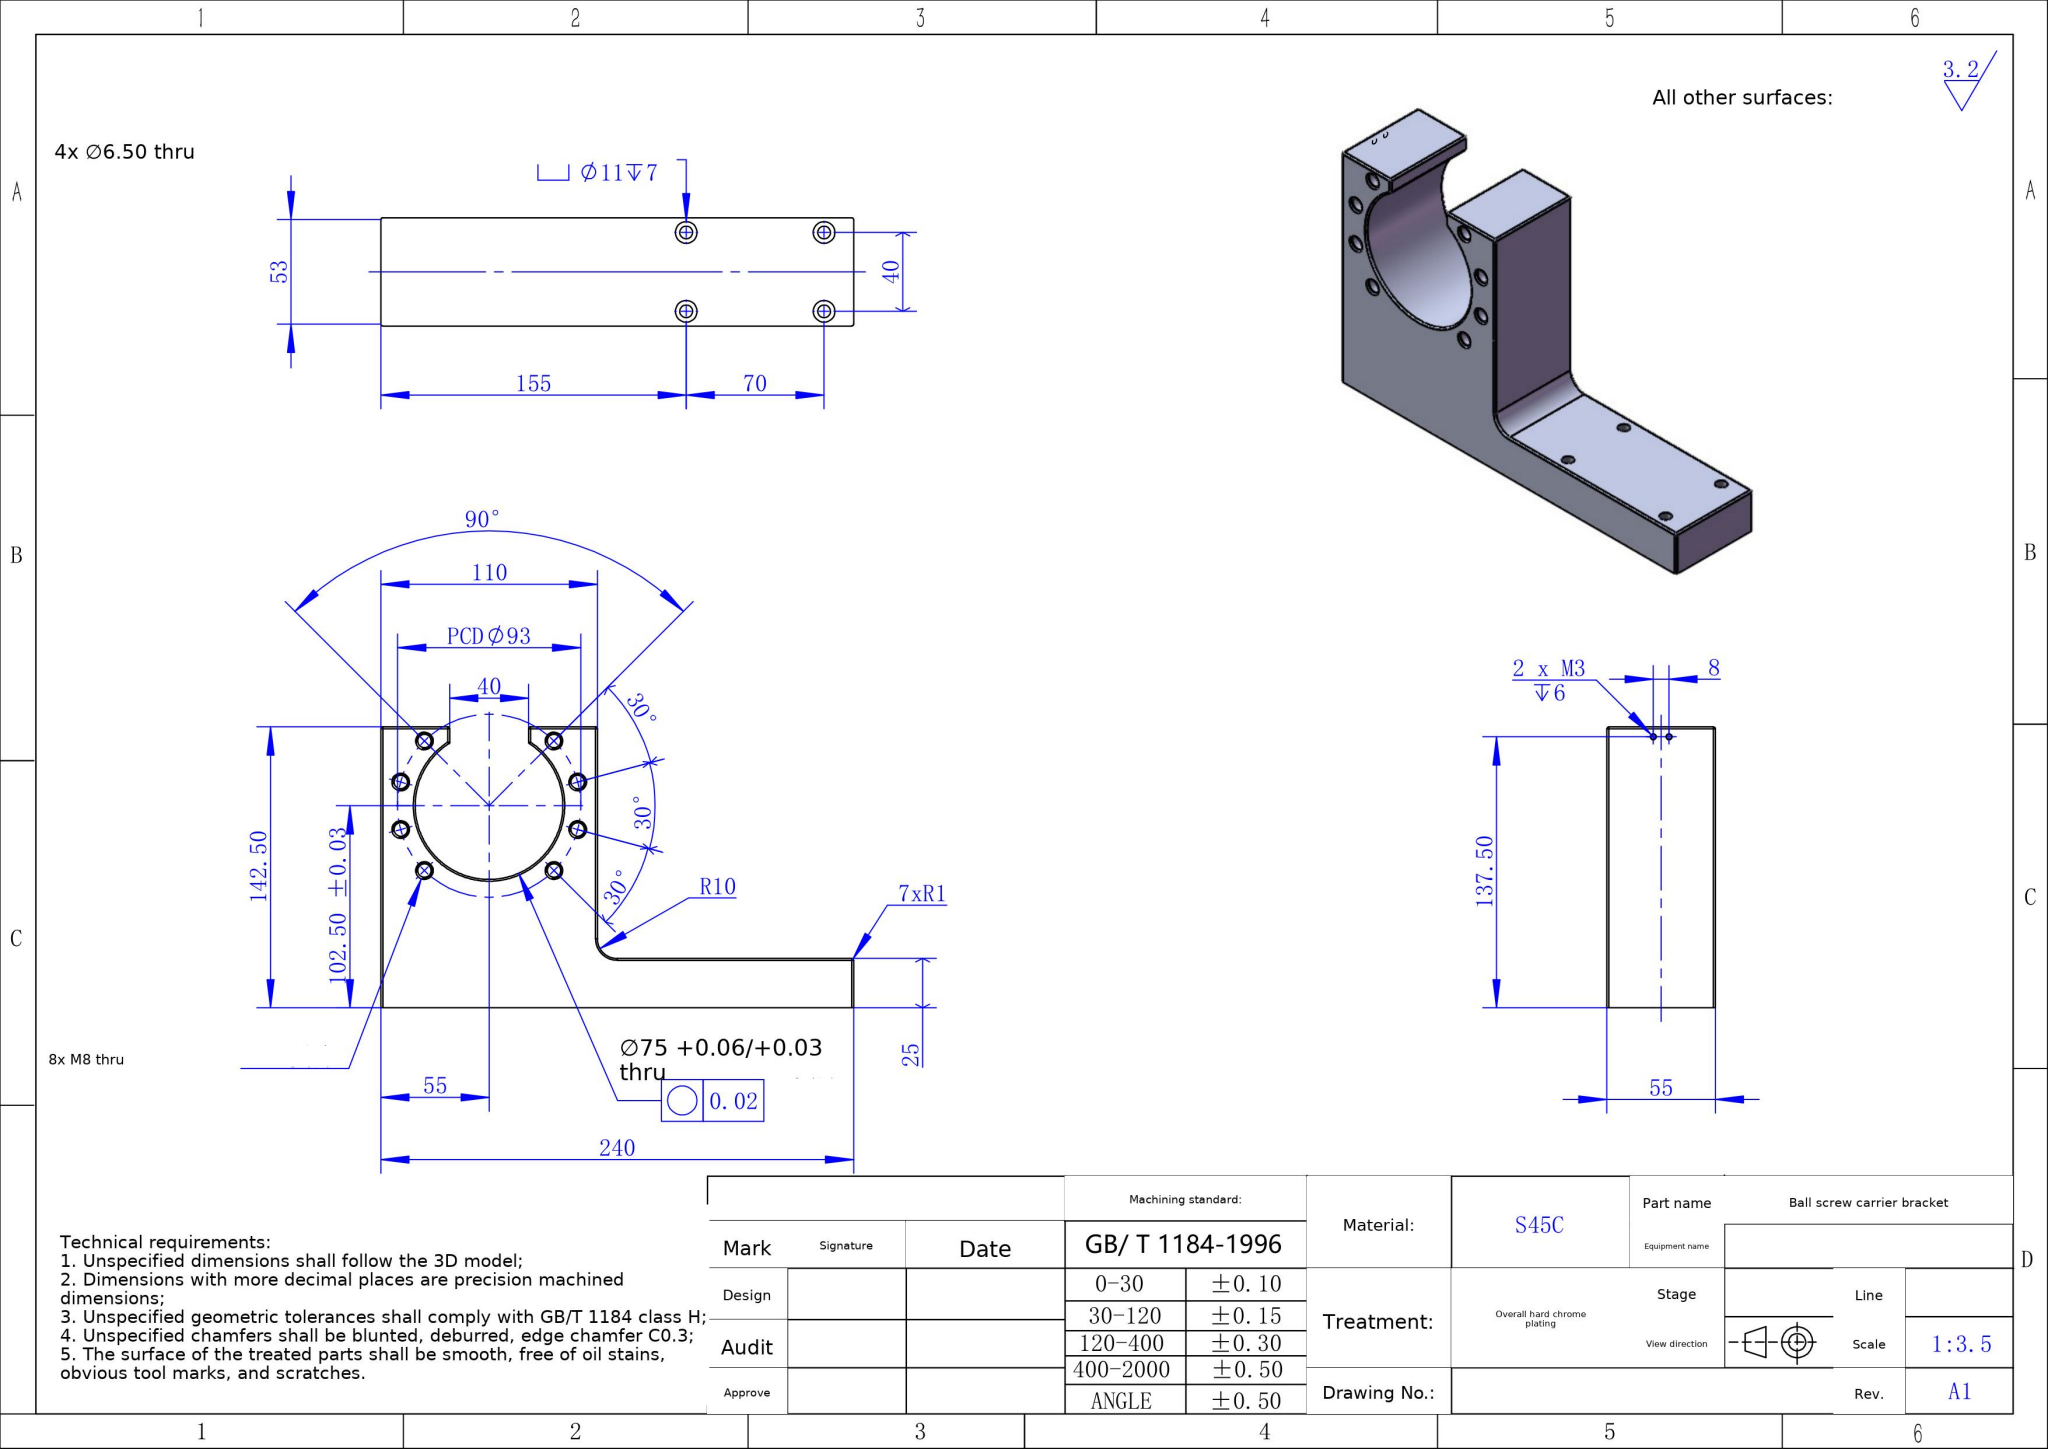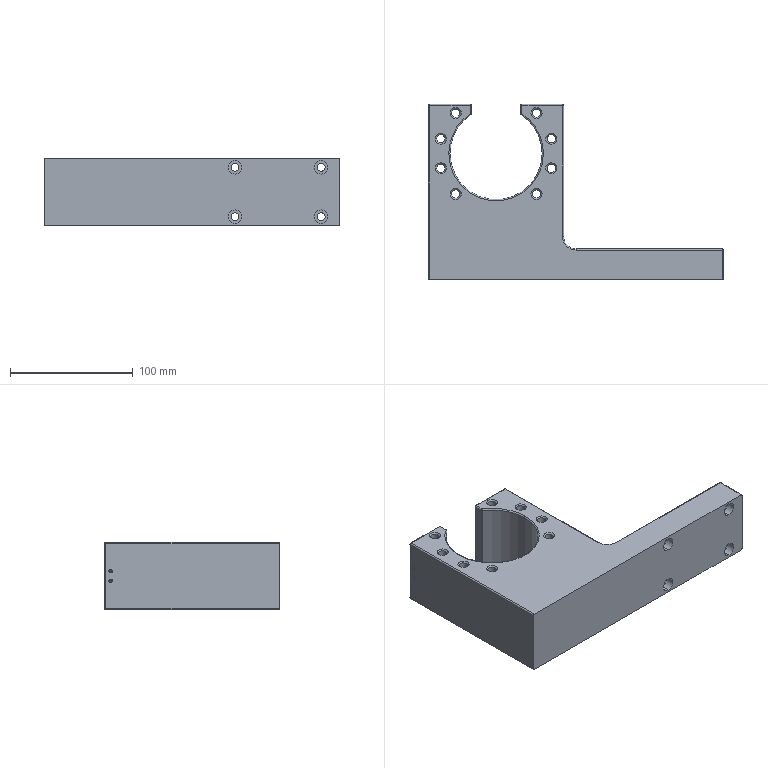Part | SolidWorks | mm | material S45C | 1 solid | 140 faces | box 240 x 142.5 x 55 mm | volume 767780 mm3 | cylinder 63 | cone 40 | plane 15 | sphere 14 | torus 8 | commonest cylinder face diameters 2 x23 6.8 x16 11 x8 6.5 x8 2.5 x4 75 x3 20 x1